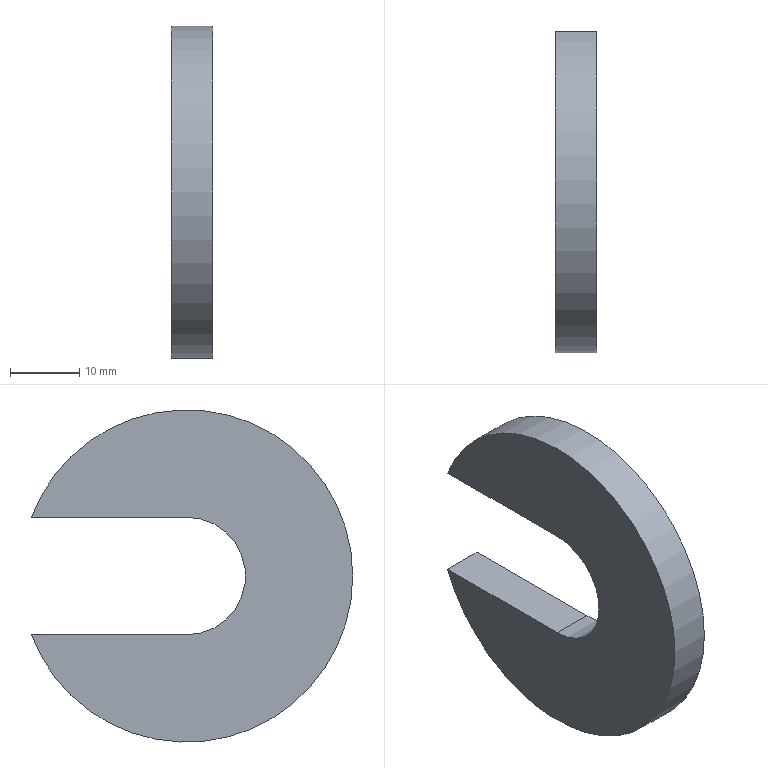Component | NX | 46_PAD_BLOCK | 1 solid | 6 faces | box 6 x 46.44 x 48 mm | volume 7781 mm3 | plane 4 | cylinder 2 | commonest cylinder face diameters 17 x1 48 x1
STEP:
#1=CARTESIAN_POINT('',(0.,0.,0.));
#2=DIRECTION('',(0.,0.,1.));
#3=DIRECTION('',(1.,0.,0.));
#4=AXIS2_PLACEMENT_3D('',#1,#2,#3);
#5=CARTESIAN_POINT('',(64.,-147.739,-18.5));
#6=VERTEX_POINT('',#5);
#7=CARTESIAN_POINT('',(58.,-147.739,-18.5));
#8=VERTEX_POINT('',#7);
#9=CARTESIAN_POINT('',(64.,-147.739,-18.5));
#10=DIRECTION('',(-1.,0.,0.));
#11=VECTOR('',#10,1.);
#12=LINE('',#9,#11);
#13=CARTESIAN_POINT('',(64.,-147.739,-10.));
#14=DIRECTION('',(-1.,0.,0.));
#15=DIRECTION('',(0.,-1.,0.));
#16=AXIS2_PLACEMENT_3D('',#13,#14,#15);
#17=CYLINDRICAL_SURFACE('',#16,8.5);
#18=CARTESIAN_POINT('',(4.712,0.));
#19=DIRECTION('',(0.,1.));
#20=VECTOR('',#19,1.);
#21=LINE('',#18,#20);
#22=(GEOMETRIC_REPRESENTATION_CONTEXT(2)PARAMETRIC_REPRESENTATION_CONTEXT()REPRESENTATION_CONTEXT('',''));
#23=DEFINITIONAL_REPRESENTATION('',(#21),#22);
#24=PCURVE('',#17,#23);
#25=CARTESIAN_POINT('',(64.,-125.295,-18.5));
#26=DIRECTION('',(0.,0.,-1.));
#27=DIRECTION('',(-1.,0.,0.));
#28=AXIS2_PLACEMENT_3D('',#25,#26,#27);
#29=PLANE('',#28);
#30=CARTESIAN_POINT('',(0.,-22.444));
#31=DIRECTION('',(1.,0.));
#32=VECTOR('',#31,1.);
#33=LINE('',#30,#32);
#34=(GEOMETRIC_REPRESENTATION_CONTEXT(2)PARAMETRIC_REPRESENTATION_CONTEXT()REPRESENTATION_CONTEXT('',''));
#35=DEFINITIONAL_REPRESENTATION('',(#33),#34);
#36=PCURVE('',#29,#35);
#37=SURFACE_CURVE('',#12,(#24,#36),.PCURVE_S1.);
#38=EDGE_CURVE('',#6,#8,#37,.T.);
#39=ORIENTED_EDGE('',*,*,#38,.F.);
#40=CARTESIAN_POINT('',(64.,-147.739,-1.5));
#41=VERTEX_POINT('',#40);
#42=CARTESIAN_POINT('',(64.,-147.739,-10.));
#43=DIRECTION('',(-1.,0.,0.));
#44=DIRECTION('',(0.,1.,0.));
#45=AXIS2_PLACEMENT_3D('',#42,#43,#44);
#46=CIRCLE('',#45,8.5);
#47=CARTESIAN_POINT('',(3.142,0.));
#48=DIRECTION('',(1.,0.));
#49=VECTOR('',#48,1.);
#50=LINE('',#47,#49);
#51=(GEOMETRIC_REPRESENTATION_CONTEXT(2)PARAMETRIC_REPRESENTATION_CONTEXT()REPRESENTATION_CONTEXT('',''));
#52=DEFINITIONAL_REPRESENTATION('',(#50),#51);
#53=PCURVE('',#17,#52);
#54=CARTESIAN_POINT('',(64.,-147.739,-10.));
#55=DIRECTION('',(-1.,0.,0.));
#56=DIRECTION('',(0.,-1.,0.));
#57=AXIS2_PLACEMENT_3D('',#54,#55,#56);
#58=PLANE('',#57);
#59=CARTESIAN_POINT('',(0.,0.));
#60=DIRECTION('',(-1.,0.));
#61=AXIS2_PLACEMENT_2D('',#59,#60);
#62=CIRCLE('',#61,8.5);
#63=(GEOMETRIC_REPRESENTATION_CONTEXT(2)PARAMETRIC_REPRESENTATION_CONTEXT()REPRESENTATION_CONTEXT('',''));
#64=DEFINITIONAL_REPRESENTATION('',(#62),#63);
#65=PCURVE('',#58,#64);
#66=SURFACE_CURVE('',#46,(#53,#65),.PCURVE_S1.);
#67=EDGE_CURVE('',#6,#41,#66,.T.);
#68=ORIENTED_EDGE('',*,*,#67,.T.);
#69=CARTESIAN_POINT('',(58.,-147.739,-1.5));
#70=VERTEX_POINT('',#69);
#71=CARTESIAN_POINT('',(64.,-147.739,-1.5));
#72=DIRECTION('',(-1.,0.,0.));
#73=VECTOR('',#72,1.);
#74=LINE('',#71,#73);
#75=CARTESIAN_POINT('',(7.854,0.));
#76=DIRECTION('',(0.,1.));
#77=VECTOR('',#76,1.);
#78=LINE('',#75,#77);
#79=(GEOMETRIC_REPRESENTATION_CONTEXT(2)PARAMETRIC_REPRESENTATION_CONTEXT()REPRESENTATION_CONTEXT('',''));
#80=DEFINITIONAL_REPRESENTATION('',(#78),#79);
#81=PCURVE('',#17,#80);
#82=CARTESIAN_POINT('',(64.,-147.739,-1.5));
#83=DIRECTION('',(0.,0.,1.));
#84=DIRECTION('',(1.,0.,0.));
#85=AXIS2_PLACEMENT_3D('',#82,#83,#84);
#86=PLANE('',#85);
#87=CARTESIAN_POINT('',(0.,0.));
#88=DIRECTION('',(-1.,0.));
#89=VECTOR('',#88,1.);
#90=LINE('',#87,#89);
#91=(GEOMETRIC_REPRESENTATION_CONTEXT(2)PARAMETRIC_REPRESENTATION_CONTEXT()REPRESENTATION_CONTEXT('',''));
#92=DEFINITIONAL_REPRESENTATION('',(#90),#91);
#93=PCURVE('',#86,#92);
#94=SURFACE_CURVE('',#74,(#81,#93),.PCURVE_S1.);
#95=EDGE_CURVE('',#41,#70,#94,.T.);
#96=ORIENTED_EDGE('',*,*,#95,.T.);
#97=CARTESIAN_POINT('',(58.,-147.739,-10.));
#98=DIRECTION('',(-1.,0.,0.));
#99=DIRECTION('',(0.,1.,0.));
#100=AXIS2_PLACEMENT_3D('',#97,#98,#99);
#101=CIRCLE('',#100,8.5);
#102=CARTESIAN_POINT('',(3.142,6.));
#103=DIRECTION('',(1.,0.));
#104=VECTOR('',#103,1.);
#105=LINE('',#102,#104);
#106=(GEOMETRIC_REPRESENTATION_CONTEXT(2)PARAMETRIC_REPRESENTATION_CONTEXT()REPRESENTATION_CONTEXT('',''));
#107=DEFINITIONAL_REPRESENTATION('',(#105),#106);
#108=PCURVE('',#17,#107);
#109=CARTESIAN_POINT('',(58.,-147.739,-10.));
#110=DIRECTION('',(-1.,0.,0.));
#111=DIRECTION('',(0.,-1.,0.));
#112=AXIS2_PLACEMENT_3D('',#109,#110,#111);
#113=PLANE('',#112);
#114=CARTESIAN_POINT('',(0.,0.));
#115=DIRECTION('',(-1.,0.));
#116=AXIS2_PLACEMENT_2D('',#114,#115);
#117=CIRCLE('',#116,8.5);
#118=(GEOMETRIC_REPRESENTATION_CONTEXT(2)PARAMETRIC_REPRESENTATION_CONTEXT()REPRESENTATION_CONTEXT('',''));
#119=DEFINITIONAL_REPRESENTATION('',(#117),#118);
#120=PCURVE('',#113,#119);
#121=SURFACE_CURVE('',#101,(#108,#120),.PCURVE_S1.);
#122=EDGE_CURVE('',#8,#70,#121,.T.);
#123=ORIENTED_EDGE('',*,*,#122,.F.);
#124=EDGE_LOOP('',(#39,#68,#96,#123));
#125=FACE_BOUND('',#124,.F.);
#126=ADVANCED_FACE('',(#125),#17,.F.);
#127=CARTESIAN_POINT('',(58.,-125.295,-1.5));
#128=VERTEX_POINT('',#127);
#129=CARTESIAN_POINT('',(58.,-147.739,-1.5));
#130=DIRECTION('',(0.,1.,0.));
#131=VECTOR('',#130,1.);
#132=LINE('',#129,#131);
#133=CARTESIAN_POINT('',(-6.,0.));
#134=DIRECTION('',(0.,1.));
#135=VECTOR('',#134,1.);
#136=LINE('',#133,#135);
#137=(GEOMETRIC_REPRESENTATION_CONTEXT(2)PARAMETRIC_REPRESENTATION_CONTEXT()REPRESENTATION_CONTEXT('',''));
#138=DEFINITIONAL_REPRESENTATION('',(#136),#137);
#139=PCURVE('',#86,#138);
#140=CARTESIAN_POINT('',(0.,8.5));
#141=DIRECTION('',(-1.,0.));
#142=VECTOR('',#141,1.);
#143=LINE('',#140,#142);
#144=(GEOMETRIC_REPRESENTATION_CONTEXT(2)PARAMETRIC_REPRESENTATION_CONTEXT()REPRESENTATION_CONTEXT('',''));
#145=DEFINITIONAL_REPRESENTATION('',(#143),#144);
#146=PCURVE('',#113,#145);
#147=SURFACE_CURVE('',#132,(#139,#146),.PCURVE_S1.);
#148=EDGE_CURVE('',#70,#128,#147,.T.);
#149=ORIENTED_EDGE('',*,*,#148,.T.);
#150=CARTESIAN_POINT('',(64.,-125.295,-1.5));
#151=VERTEX_POINT('',#150);
#152=CARTESIAN_POINT('',(64.,-125.295,-1.5));
#153=DIRECTION('',(-1.,0.,0.));
#154=VECTOR('',#153,1.);
#155=LINE('',#152,#154);
#156=CARTESIAN_POINT('',(0.,22.444));
#157=DIRECTION('',(-1.,0.));
#158=VECTOR('',#157,1.);
#159=LINE('',#156,#158);
#160=(GEOMETRIC_REPRESENTATION_CONTEXT(2)PARAMETRIC_REPRESENTATION_CONTEXT()REPRESENTATION_CONTEXT('',''));
#161=DEFINITIONAL_REPRESENTATION('',(#159),#160);
#162=PCURVE('',#86,#161);
#163=CARTESIAN_POINT('',(64.,-147.739,-10.));
#164=DIRECTION('',(-1.,0.,0.));
#165=DIRECTION('',(0.,-1.,0.));
#166=AXIS2_PLACEMENT_3D('',#163,#164,#165);
#167=CYLINDRICAL_SURFACE('',#166,24.);
#168=CARTESIAN_POINT('',(2.78,0.));
#169=DIRECTION('',(0.,1.));
#170=VECTOR('',#169,1.);
#171=LINE('',#168,#170);
#172=(GEOMETRIC_REPRESENTATION_CONTEXT(2)PARAMETRIC_REPRESENTATION_CONTEXT()REPRESENTATION_CONTEXT('',''));
#173=DEFINITIONAL_REPRESENTATION('',(#171),#172);
#174=PCURVE('',#167,#173);
#175=SURFACE_CURVE('',#155,(#162,#174),.PCURVE_S1.);
#176=EDGE_CURVE('',#151,#128,#175,.T.);
#177=ORIENTED_EDGE('',*,*,#176,.F.);
#178=CARTESIAN_POINT('',(64.,-147.739,-1.5));
#179=DIRECTION('',(0.,1.,0.));
#180=VECTOR('',#179,1.);
#181=LINE('',#178,#180);
#182=CARTESIAN_POINT('',(0.,0.));
#183=DIRECTION('',(0.,1.));
#184=VECTOR('',#183,1.);
#185=LINE('',#182,#184);
#186=(GEOMETRIC_REPRESENTATION_CONTEXT(2)PARAMETRIC_REPRESENTATION_CONTEXT()REPRESENTATION_CONTEXT('',''));
#187=DEFINITIONAL_REPRESENTATION('',(#185),#186);
#188=PCURVE('',#86,#187);
#189=CARTESIAN_POINT('',(0.,8.5));
#190=DIRECTION('',(-1.,0.));
#191=VECTOR('',#190,1.);
#192=LINE('',#189,#191);
#193=(GEOMETRIC_REPRESENTATION_CONTEXT(2)PARAMETRIC_REPRESENTATION_CONTEXT()REPRESENTATION_CONTEXT('',''));
#194=DEFINITIONAL_REPRESENTATION('',(#192),#193);
#195=PCURVE('',#58,#194);
#196=SURFACE_CURVE('',#181,(#188,#195),.PCURVE_S1.);
#197=EDGE_CURVE('',#41,#151,#196,.T.);
#198=ORIENTED_EDGE('',*,*,#197,.F.);
#199=ORIENTED_EDGE('',*,*,#95,.T.);
#200=EDGE_LOOP('',(#149,#177,#198,#199));
#201=FACE_BOUND('',#200,.T.);
#202=ADVANCED_FACE('',(#201),#86,.F.);
#203=CARTESIAN_POINT('',(58.,-125.295,-18.5));
#204=VERTEX_POINT('',#203);
#205=CARTESIAN_POINT('',(58.,-147.739,-10.));
#206=DIRECTION('',(1.,0.,0.));
#207=DIRECTION('',(0.,1.,0.));
#208=AXIS2_PLACEMENT_3D('',#205,#206,#207);
#209=CIRCLE('',#208,24.);
#210=CARTESIAN_POINT('',(3.142,6.));
#211=DIRECTION('',(-1.,0.));
#212=VECTOR('',#211,1.);
#213=LINE('',#210,#212);
#214=(GEOMETRIC_REPRESENTATION_CONTEXT(2)PARAMETRIC_REPRESENTATION_CONTEXT()REPRESENTATION_CONTEXT('',''));
#215=DEFINITIONAL_REPRESENTATION('',(#213),#214);
#216=PCURVE('',#167,#215);
#217=CARTESIAN_POINT('',(-24.,0.));
#218=CARTESIAN_POINT('',(-24.,41.569));
#219=CARTESIAN_POINT('',(12.,20.785));
#220=CARTESIAN_POINT('',(48.,0.));
#221=CARTESIAN_POINT('',(12.,-20.785));
#222=CARTESIAN_POINT('',(-24.,-41.569));
#223=CARTESIAN_POINT('',(-24.,0.));
#224=(BOUNDED_CURVE()B_SPLINE_CURVE(2,(#217,#218,#219,#220,#221,#222,#223),.UNSPECIFIED.,.T.,.F.)B_SPLINE_CURVE_WITH_KNOTS((1,2,2,2,2,1),(-2.094,0.,2.094,4.189,6.283,8.378),.UNSPECIFIED.)CURVE()GEOMETRIC_REPRESENTATION_ITEM()RATIONAL_B_SPLINE_CURVE((1.,0.5,1.,0.5,1.,0.5,1.))REPRESENTATION_ITEM(''));
#225=(GEOMETRIC_REPRESENTATION_CONTEXT(2)PARAMETRIC_REPRESENTATION_CONTEXT()REPRESENTATION_CONTEXT('',''));
#226=DEFINITIONAL_REPRESENTATION('',(#224),#225);
#227=PCURVE('',#113,#226);
#228=SURFACE_CURVE('',#209,(#216,#227),.PCURVE_S1.);
#229=EDGE_CURVE('',#128,#204,#228,.T.);
#230=ORIENTED_EDGE('',*,*,#229,.T.);
#231=CARTESIAN_POINT('',(64.,-125.295,-18.5));
#232=VERTEX_POINT('',#231);
#233=CARTESIAN_POINT('',(64.,-125.295,-18.5));
#234=DIRECTION('',(-1.,0.,0.));
#235=VECTOR('',#234,1.);
#236=LINE('',#233,#235);
#237=CARTESIAN_POINT('',(-2.78,0.));
#238=DIRECTION('',(0.,1.));
#239=VECTOR('',#238,1.);
#240=LINE('',#237,#239);
#241=(GEOMETRIC_REPRESENTATION_CONTEXT(2)PARAMETRIC_REPRESENTATION_CONTEXT()REPRESENTATION_CONTEXT('',''));
#242=DEFINITIONAL_REPRESENTATION('',(#240),#241);
#243=PCURVE('',#167,#242);
#244=CARTESIAN_POINT('',(0.,0.));
#245=DIRECTION('',(1.,0.));
#246=VECTOR('',#245,1.);
#247=LINE('',#244,#246);
#248=(GEOMETRIC_REPRESENTATION_CONTEXT(2)PARAMETRIC_REPRESENTATION_CONTEXT()REPRESENTATION_CONTEXT('',''));
#249=DEFINITIONAL_REPRESENTATION('',(#247),#248);
#250=PCURVE('',#29,#249);
#251=SURFACE_CURVE('',#236,(#243,#250),.PCURVE_S1.);
#252=EDGE_CURVE('',#232,#204,#251,.T.);
#253=ORIENTED_EDGE('',*,*,#252,.F.);
#254=CARTESIAN_POINT('',(64.,-147.739,-10.));
#255=DIRECTION('',(1.,0.,0.));
#256=DIRECTION('',(0.,1.,0.));
#257=AXIS2_PLACEMENT_3D('',#254,#255,#256);
#258=CIRCLE('',#257,24.);
#259=CARTESIAN_POINT('',(3.142,0.));
#260=DIRECTION('',(-1.,0.));
#261=VECTOR('',#260,1.);
#262=LINE('',#259,#261);
#263=(GEOMETRIC_REPRESENTATION_CONTEXT(2)PARAMETRIC_REPRESENTATION_CONTEXT()REPRESENTATION_CONTEXT('',''));
#264=DEFINITIONAL_REPRESENTATION('',(#262),#263);
#265=PCURVE('',#167,#264);
#266=CARTESIAN_POINT('',(-24.,0.));
#267=CARTESIAN_POINT('',(-24.,41.569));
#268=CARTESIAN_POINT('',(12.,20.785));
#269=CARTESIAN_POINT('',(48.,0.));
#270=CARTESIAN_POINT('',(12.,-20.785));
#271=CARTESIAN_POINT('',(-24.,-41.569));
#272=CARTESIAN_POINT('',(-24.,0.));
#273=(BOUNDED_CURVE()B_SPLINE_CURVE(2,(#266,#267,#268,#269,#270,#271,#272),.UNSPECIFIED.,.T.,.F.)B_SPLINE_CURVE_WITH_KNOTS((1,2,2,2,2,1),(-2.094,0.,2.094,4.189,6.283,8.378),.UNSPECIFIED.)CURVE()GEOMETRIC_REPRESENTATION_ITEM()RATIONAL_B_SPLINE_CURVE((1.,0.5,1.,0.5,1.,0.5,1.))REPRESENTATION_ITEM(''));
#274=(GEOMETRIC_REPRESENTATION_CONTEXT(2)PARAMETRIC_REPRESENTATION_CONTEXT()REPRESENTATION_CONTEXT('',''));
#275=DEFINITIONAL_REPRESENTATION('',(#273),#274);
#276=PCURVE('',#58,#275);
#277=SURFACE_CURVE('',#258,(#265,#276),.PCURVE_S1.);
#278=EDGE_CURVE('',#151,#232,#277,.T.);
#279=ORIENTED_EDGE('',*,*,#278,.F.);
#280=ORIENTED_EDGE('',*,*,#176,.T.);
#281=EDGE_LOOP('',(#230,#253,#279,#280));
#282=FACE_BOUND('',#281,.T.);
#283=ADVANCED_FACE('',(#282),#167,.T.);
#284=CARTESIAN_POINT('',(58.,-125.295,-18.5));
#285=DIRECTION('',(0.,-1.,0.));
#286=VECTOR('',#285,1.);
#287=LINE('',#284,#286);
#288=CARTESIAN_POINT('',(6.,0.));
#289=DIRECTION('',(0.,-1.));
#290=VECTOR('',#289,1.);
#291=LINE('',#288,#290);
#292=(GEOMETRIC_REPRESENTATION_CONTEXT(2)PARAMETRIC_REPRESENTATION_CONTEXT()REPRESENTATION_CONTEXT('',''));
#293=DEFINITIONAL_REPRESENTATION('',(#291),#292);
#294=PCURVE('',#29,#293);
#295=CARTESIAN_POINT('',(-22.444,-8.5));
#296=DIRECTION('',(1.,0.));
#297=VECTOR('',#296,1.);
#298=LINE('',#295,#297);
#299=(GEOMETRIC_REPRESENTATION_CONTEXT(2)PARAMETRIC_REPRESENTATION_CONTEXT()REPRESENTATION_CONTEXT('',''));
#300=DEFINITIONAL_REPRESENTATION('',(#298),#299);
#301=PCURVE('',#113,#300);
#302=SURFACE_CURVE('',#287,(#294,#301),.PCURVE_S1.);
#303=EDGE_CURVE('',#204,#8,#302,.T.);
#304=ORIENTED_EDGE('',*,*,#303,.T.);
#305=ORIENTED_EDGE('',*,*,#38,.F.);
#306=CARTESIAN_POINT('',(64.,-125.295,-18.5));
#307=DIRECTION('',(0.,-1.,0.));
#308=VECTOR('',#307,1.);
#309=LINE('',#306,#308);
#310=CARTESIAN_POINT('',(0.,0.));
#311=DIRECTION('',(0.,-1.));
#312=VECTOR('',#311,1.);
#313=LINE('',#310,#312);
#314=(GEOMETRIC_REPRESENTATION_CONTEXT(2)PARAMETRIC_REPRESENTATION_CONTEXT()REPRESENTATION_CONTEXT('',''));
#315=DEFINITIONAL_REPRESENTATION('',(#313),#314);
#316=PCURVE('',#29,#315);
#317=CARTESIAN_POINT('',(-22.444,-8.5));
#318=DIRECTION('',(1.,0.));
#319=VECTOR('',#318,1.);
#320=LINE('',#317,#319);
#321=(GEOMETRIC_REPRESENTATION_CONTEXT(2)PARAMETRIC_REPRESENTATION_CONTEXT()REPRESENTATION_CONTEXT('',''));
#322=DEFINITIONAL_REPRESENTATION('',(#320),#321);
#323=PCURVE('',#58,#322);
#324=SURFACE_CURVE('',#309,(#316,#323),.PCURVE_S1.);
#325=EDGE_CURVE('',#232,#6,#324,.T.);
#326=ORIENTED_EDGE('',*,*,#325,.F.);
#327=ORIENTED_EDGE('',*,*,#252,.T.);
#328=EDGE_LOOP('',(#304,#305,#326,#327));
#329=FACE_BOUND('',#328,.T.);
#330=ADVANCED_FACE('',(#329),#29,.F.);
#331=ORIENTED_EDGE('',*,*,#67,.T.);
#332=ORIENTED_EDGE('',*,*,#197,.T.);
#333=ORIENTED_EDGE('',*,*,#278,.T.);
#334=ORIENTED_EDGE('',*,*,#325,.T.);
#335=EDGE_LOOP('',(#331,#332,#333,#334));
#336=FACE_BOUND('',#335,.T.);
#337=ADVANCED_FACE('',(#336),#58,.F.);
#338=ORIENTED_EDGE('',*,*,#122,.F.);
#339=ORIENTED_EDGE('',*,*,#303,.F.);
#340=ORIENTED_EDGE('',*,*,#229,.F.);
#341=ORIENTED_EDGE('',*,*,#148,.F.);
#342=EDGE_LOOP('',(#338,#339,#340,#341));
#343=FACE_BOUND('',#342,.T.);
#344=ADVANCED_FACE('',(#343),#113,.T.);
#345=CLOSED_SHELL('',(#126,#202,#283,#330,#337,#344));
#346=MANIFOLD_SOLID_BREP('',#345);
#347=(LENGTH_UNIT()NAMED_UNIT(*)SI_UNIT(.MILLI.,.METRE.));
#348=UNCERTAINTY_MEASURE_WITH_UNIT(LENGTH_MEASURE(0.0000001),#347,'','');
#349=(NAMED_UNIT(*)PLANE_ANGLE_UNIT()SI_UNIT($,.RADIAN.));
#350=(NAMED_UNIT(*)SI_UNIT($,.STERADIAN.)SOLID_ANGLE_UNIT());
#351=(GEOMETRIC_REPRESENTATION_CONTEXT(3)GLOBAL_UNCERTAINTY_ASSIGNED_CONTEXT((#348))GLOBAL_UNIT_ASSIGNED_CONTEXT((#347,#349,#350))REPRESENTATION_CONTEXT('',''));
#352=ADVANCED_BREP_SHAPE_REPRESENTATION('',(#4,#346),#351);